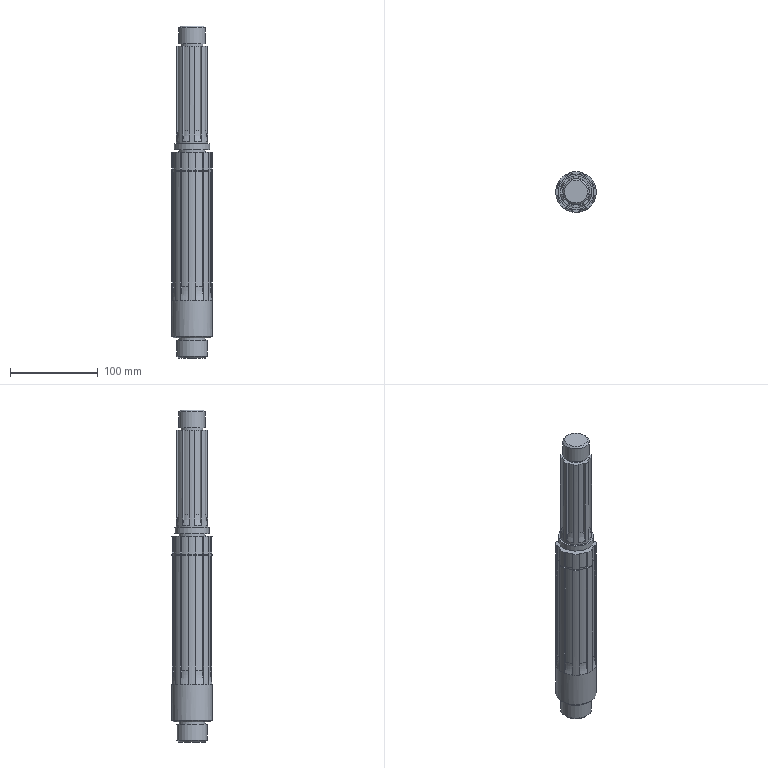Component | NX | Root-owned geometry | 3 solids | 159 faces | volume 477059 mm3 | plane 91 | cylinder 49 | torus 16 | cone 3 | commonest cylinder face diameters 46 x17 42.5 x16 32 x8 30 x3 36 x1 40 x1 35 x1 43 x1